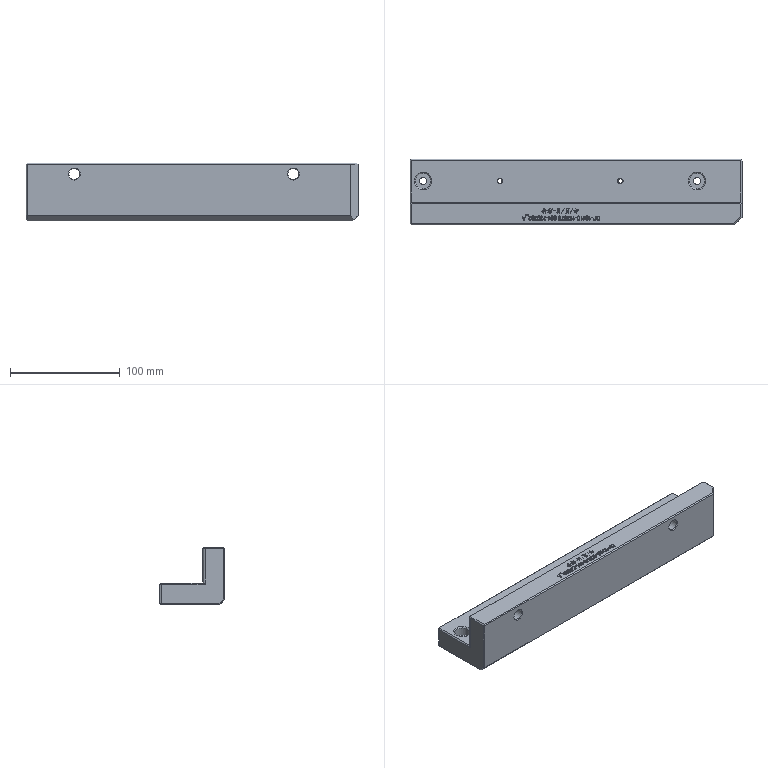CAM job | NX | mm | 3-axis | 5 set-ups | 49 operations | part box 303 x 60 x 52.8
set-up 1
1. Face Milling | Mill Mill5 E50R0.8 | FACE_MILLING_1 | path 4388.2 mm | 5.098 min
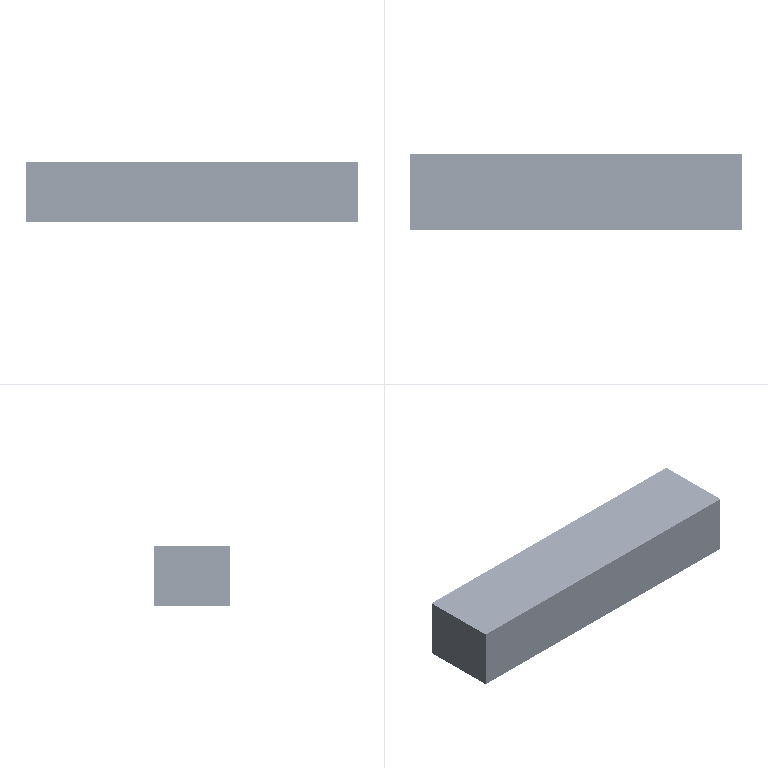2. Planar Roughing | Mill Mill5 LX-D12 | PLANAR_ROUGHING_2 | path 55757.865 mm | 27.343 min
3. Planar Milling | Mill Mill5 LX-D12J | PLANAR_MILLING_3 | path 8035.48 mm | 3.971 min
set-up 2
4. Face Milling | Mill Mill5 E50R0.8 | FACE_MILLING_4 | path 4323.2 mm | 2.03 min
5. Planar Roughing | Mill Mill5 LX-D10 | PLANAR_ROUGHING_5 | path 26148.432 mm | 9.637 min
6. Drilling | Mill MillChamfer DXZ-D10A90 | DRILLING_6 | path 344 mm | 0.1136 min
7. Drilling | Mill MillChamfer DXZ-D10A90 | DRILLING_7 | path 204 mm | 0.0996 min
8. Drilling | Drill DrillStandard ZT-D6.3 | DRILLING_8 | path 780.069 mm | 0.9893 min
9. Drilling | Drill DrillStandard ZT-D3.8 | DRILLING_9 | path 1350.798 mm | 0.9453 min
10. Cylinder Milling | Mill Mill5 LX-D6 | CYLINDER_MILLING_10 | path 980.438 mm | 0.9708 min
11. Face Milling | Mill Mill5 E50R0.8 | FACE_MILLING_11 | path 842.667 mm | 1.003 min
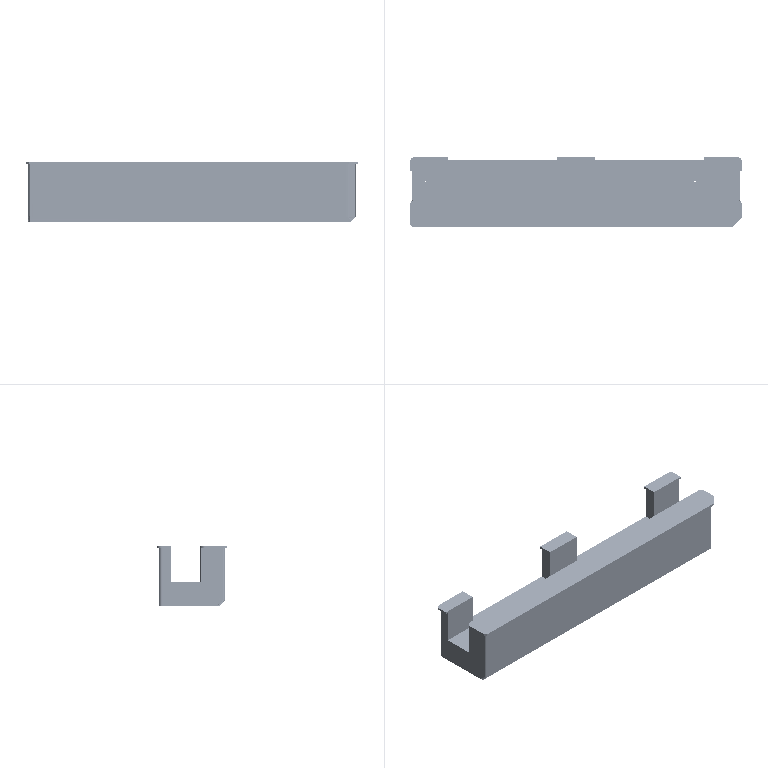12. Cylinder Milling | Mill Mill5 LX-D6J | CYLINDER_MILLING_12 | path 1610.966 mm | 3.496 min
13. Cylinder Milling | Mill Mill5 LX-D4J | CYLINDER_MILLING_13 | path 780.196 mm | 1.094 min
14. Cylinder Milling | Mill Mill5 LX-D3J | CYLINDER_MILLING_14 | path 416.84 mm | 0.4 min
15. Planar Milling | Mill Mill5 LX-D16J | PLANAR_MILLING_15 | path 3356.811 mm | 3.921 min
16. Fixed-axis Surface Contouring | Mill MillChamfer DJ-D10A90 | FIXED-AXIS_SURFACE_CONTOURING_16 | path 371.214 mm | 0.1262 min
17. Volume Based 2.5D Milling | Mill MillChamfer DJ-D10A90 | VOLUME_BASED_2.5D_MILLING_17 | path 264.24 mm | 0.1416 min
18. Volume Based 2.5D Milling | Mill MillChamfer DJ-D10A90 | VOLUME_BASED_2.5D_MILLING_18 | path 411.754 mm | 0.7304 min
19. Z-Level Milling | Mill Mill5 YB-D10R1 | Z-LEVEL_MILLING_19 | path 3286.501 mm | 1.623 min
20. Z-Level Milling | Mill Mill5 YB-D10R1 | Z-LEVEL_MILLING_20 | path 17178.095 mm | 8.571 min
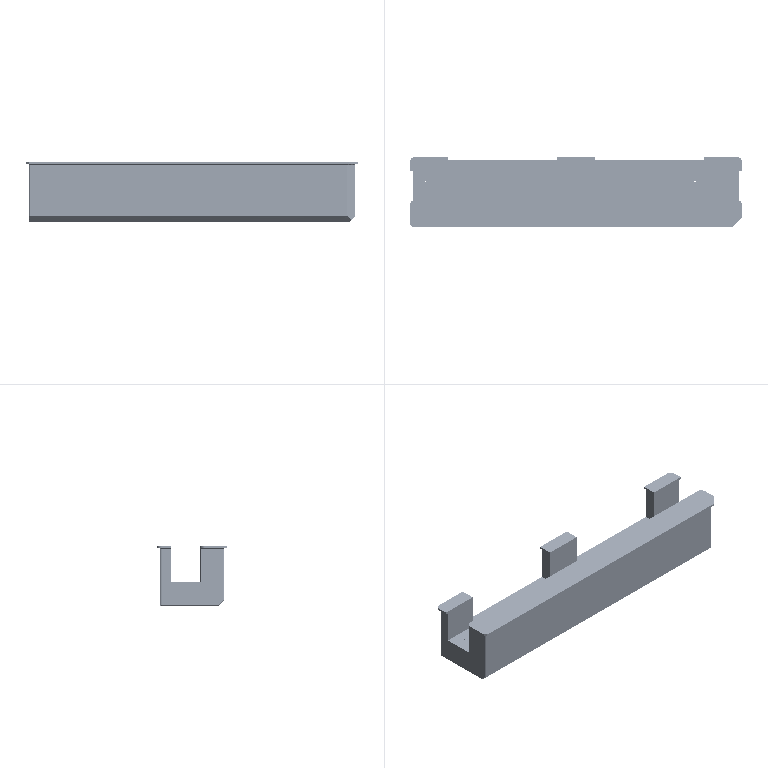21. Planar Milling | Mill Mill5 LX-D12J | PLANAR_MILLING_21 | path 8139.435 mm | 4.046 min
set-up 3
22. Face Milling | Mill Mill5 E50R0.8 | FACE_MILLING_22 | path 2580.133 mm | 1.216 min
23. Cavity Milling | Mill Mill5 LX-D12 | CAVITY_MILLING_23 | path 71660.269 mm | 15.05 min
24. Cylinder Milling | Mill Mill5 LX-D8 | CYLINDER_MILLING_24 | path 1231.419 mm | 0.9904 min
25. Volume Based 2.5D Milling | Mill Mill5 LX-D12J | VOLUME_BASED_2.5D_MILLING_25 | path 1072.606 mm | 1.23 min
26. Volume Based 2.5D Milling | Mill Mill5 LX-D12J | VOLUME_BASED_2.5D_MILLING_26 | path 2109.319 mm | 2.453 min
27. Volume Based 2.5D Milling | Mill Mill5 LX-D12J | VOLUME_BASED_2.5D_MILLING_27 | path 2063.803 mm | 1.354 min
28. Cylinder Milling | Mill Mill5 LX-D8J | CYLINDER_MILLING_28 | path 923.195 mm | 1.162 min
29. Volume Based 2.5D Milling | Mill MillChamfer DJ-D10A90 | VOLUME_BASED_2.5D_MILLING_29 | path 706.46 mm | 0.8267 min
30. Volume Based 2.5D Milling | Mill MillChamfer DJ-D10A90 | VOLUME_BASED_2.5D_MILLING_30 | path 570.035 mm | 0.1555 min
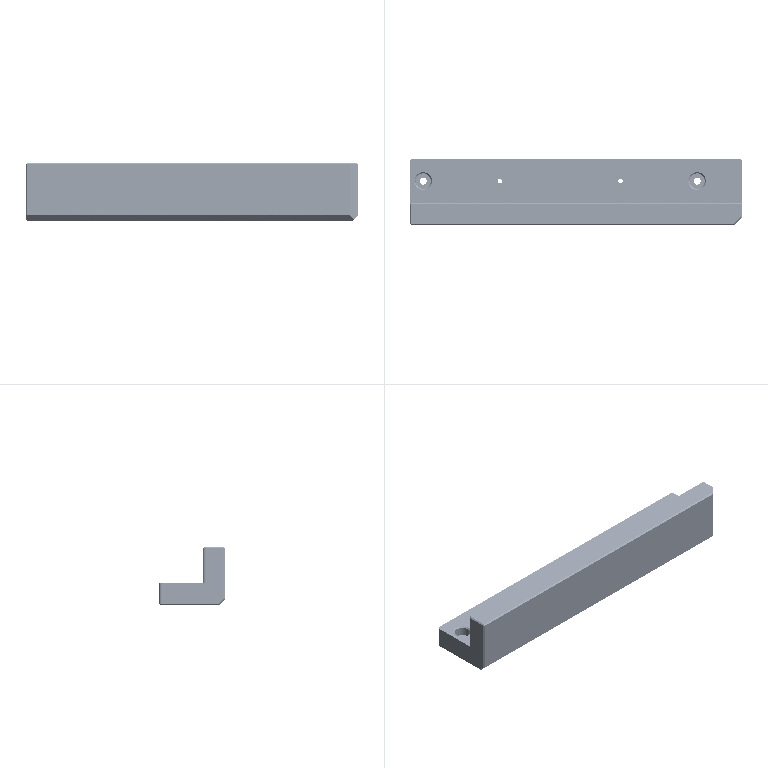31. Drilling | Mill MillChamfer DJ-D10A90 | DRILLING_31 | path 341.2 mm | 0.1077 min
32. Volume Based 2.5D Milling | Mill MillChamfer DJ-D6A90 | VOLUME_BASED_2.5D_MILLING_32 | path 1343.458 mm | 1.085 min
33. Planar Text | Mill Mill5 KZ-D0.5R0.25 | PLANAR_TEXT_33 | path 21108.856 mm | 5.329 min
34. Planar Milling | Mill Mill5 LX-D12J | PLANAR_MILLING_34 | path 8169.516 mm | 4.056 min
set-up 4
35. Cavity Milling | Mill Mill5 LX-D8 | CAVITY_MILLING_35 | path 6105.895 mm | 4.186 min
36. Cylinder Milling | Mill Mill5 LX-D8 | CYLINDER_MILLING_36 | path 850.489 mm | 0.4993 min
37. Cylinder Milling | Mill Mill5 LX-D8J | CYLINDER_MILLING_37 | path 1084.11 mm | 1.662 min
38. Planar Milling | Mill Mill5 LX-D8J | PLANAR_MILLING_38 | path 578.753 mm | 0.1895 min
39. Cylinder Milling | Mill Mill5 LX-D8J | CYLINDER_MILLING_39 | path 685.386 mm | 0.5381 min
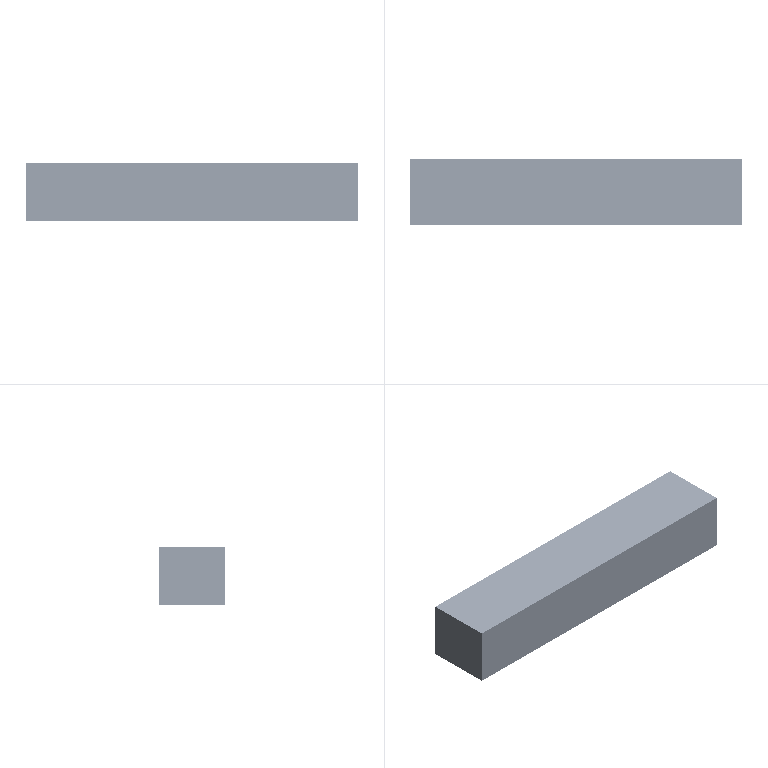40. Cavity Milling | Mill Mill5 LX-D4J | CAVITY_MILLING_40 | path 1392.761 mm | 0.3674 min
41. Volume Based 2.5D Milling | Mill MillChamfer DJ-D10A90 | VOLUME_BASED_2.5D_MILLING_41 | path 584.173 mm | 0.2224 min
42. Volume Based 2.5D Milling | Mill MillChamfer DJ-D10A90 | VOLUME_BASED_2.5D_MILLING_42 | path 532.239 mm | 0.1229 min
43. Drilling | Mill MillChamfer DXZ-D4A90 | DRILLING_43 | path 474 mm | 0.1266 min
44. Drilling | Drill DrillStandard ZT-D3.3 | DRILLING_44 | path 1059.605 mm | 0.5263 min
45. Cylinder Milling | Mill Mill5 LX-D3J | CYLINDER_MILLING_45 | path 592.991 mm | 0.3149 min
46. Volume Based 2.5D Milling | Mill MillChamfer DJ-D4A90 | VOLUME_BASED_2.5D_MILLING_46 | path 598.946 mm | 0.2109 min
47. Thread Milling | Drill DrillThreadMill M4X0.7-D3.15 | THREAD_MILLING_47 | path 708.308 mm | 0.4167 min
48. Thread Milling | Drill DrillThreadMill M4X0.7-D3.15 | THREAD_MILLING_48 | path 566.702 mm | 0.2104 min
set-up 5
49. Volume Based 2.5D Milling | Mill MillChamfer DJ-D10A90 | VOLUME_BASED_2.5D_MILLING_49 | path 350.924 mm | 0.1048 min